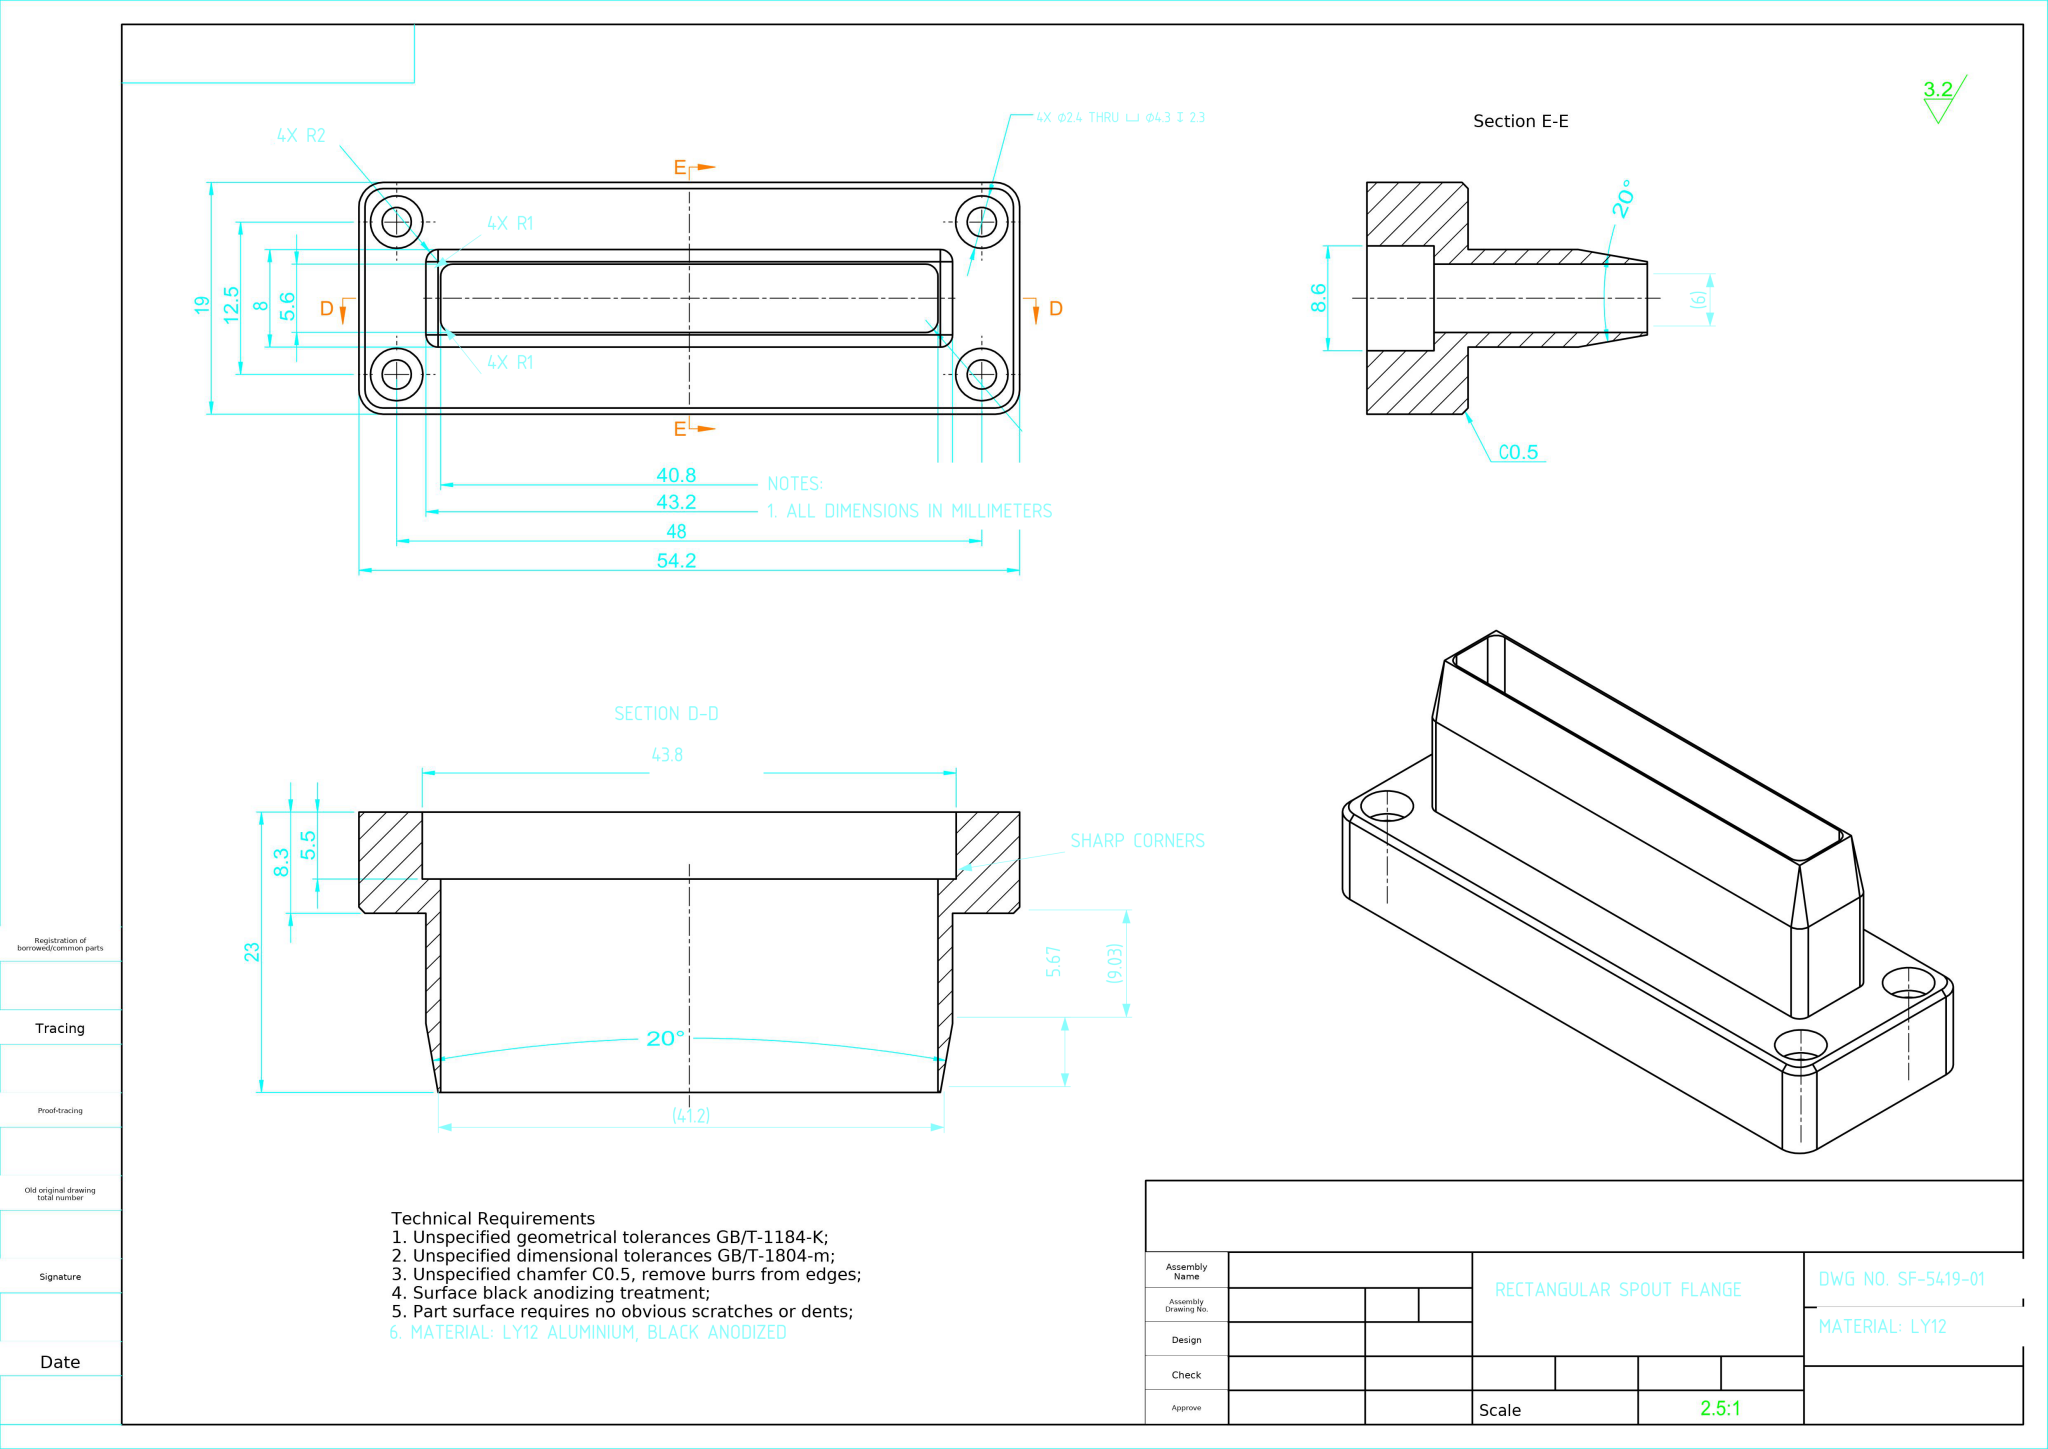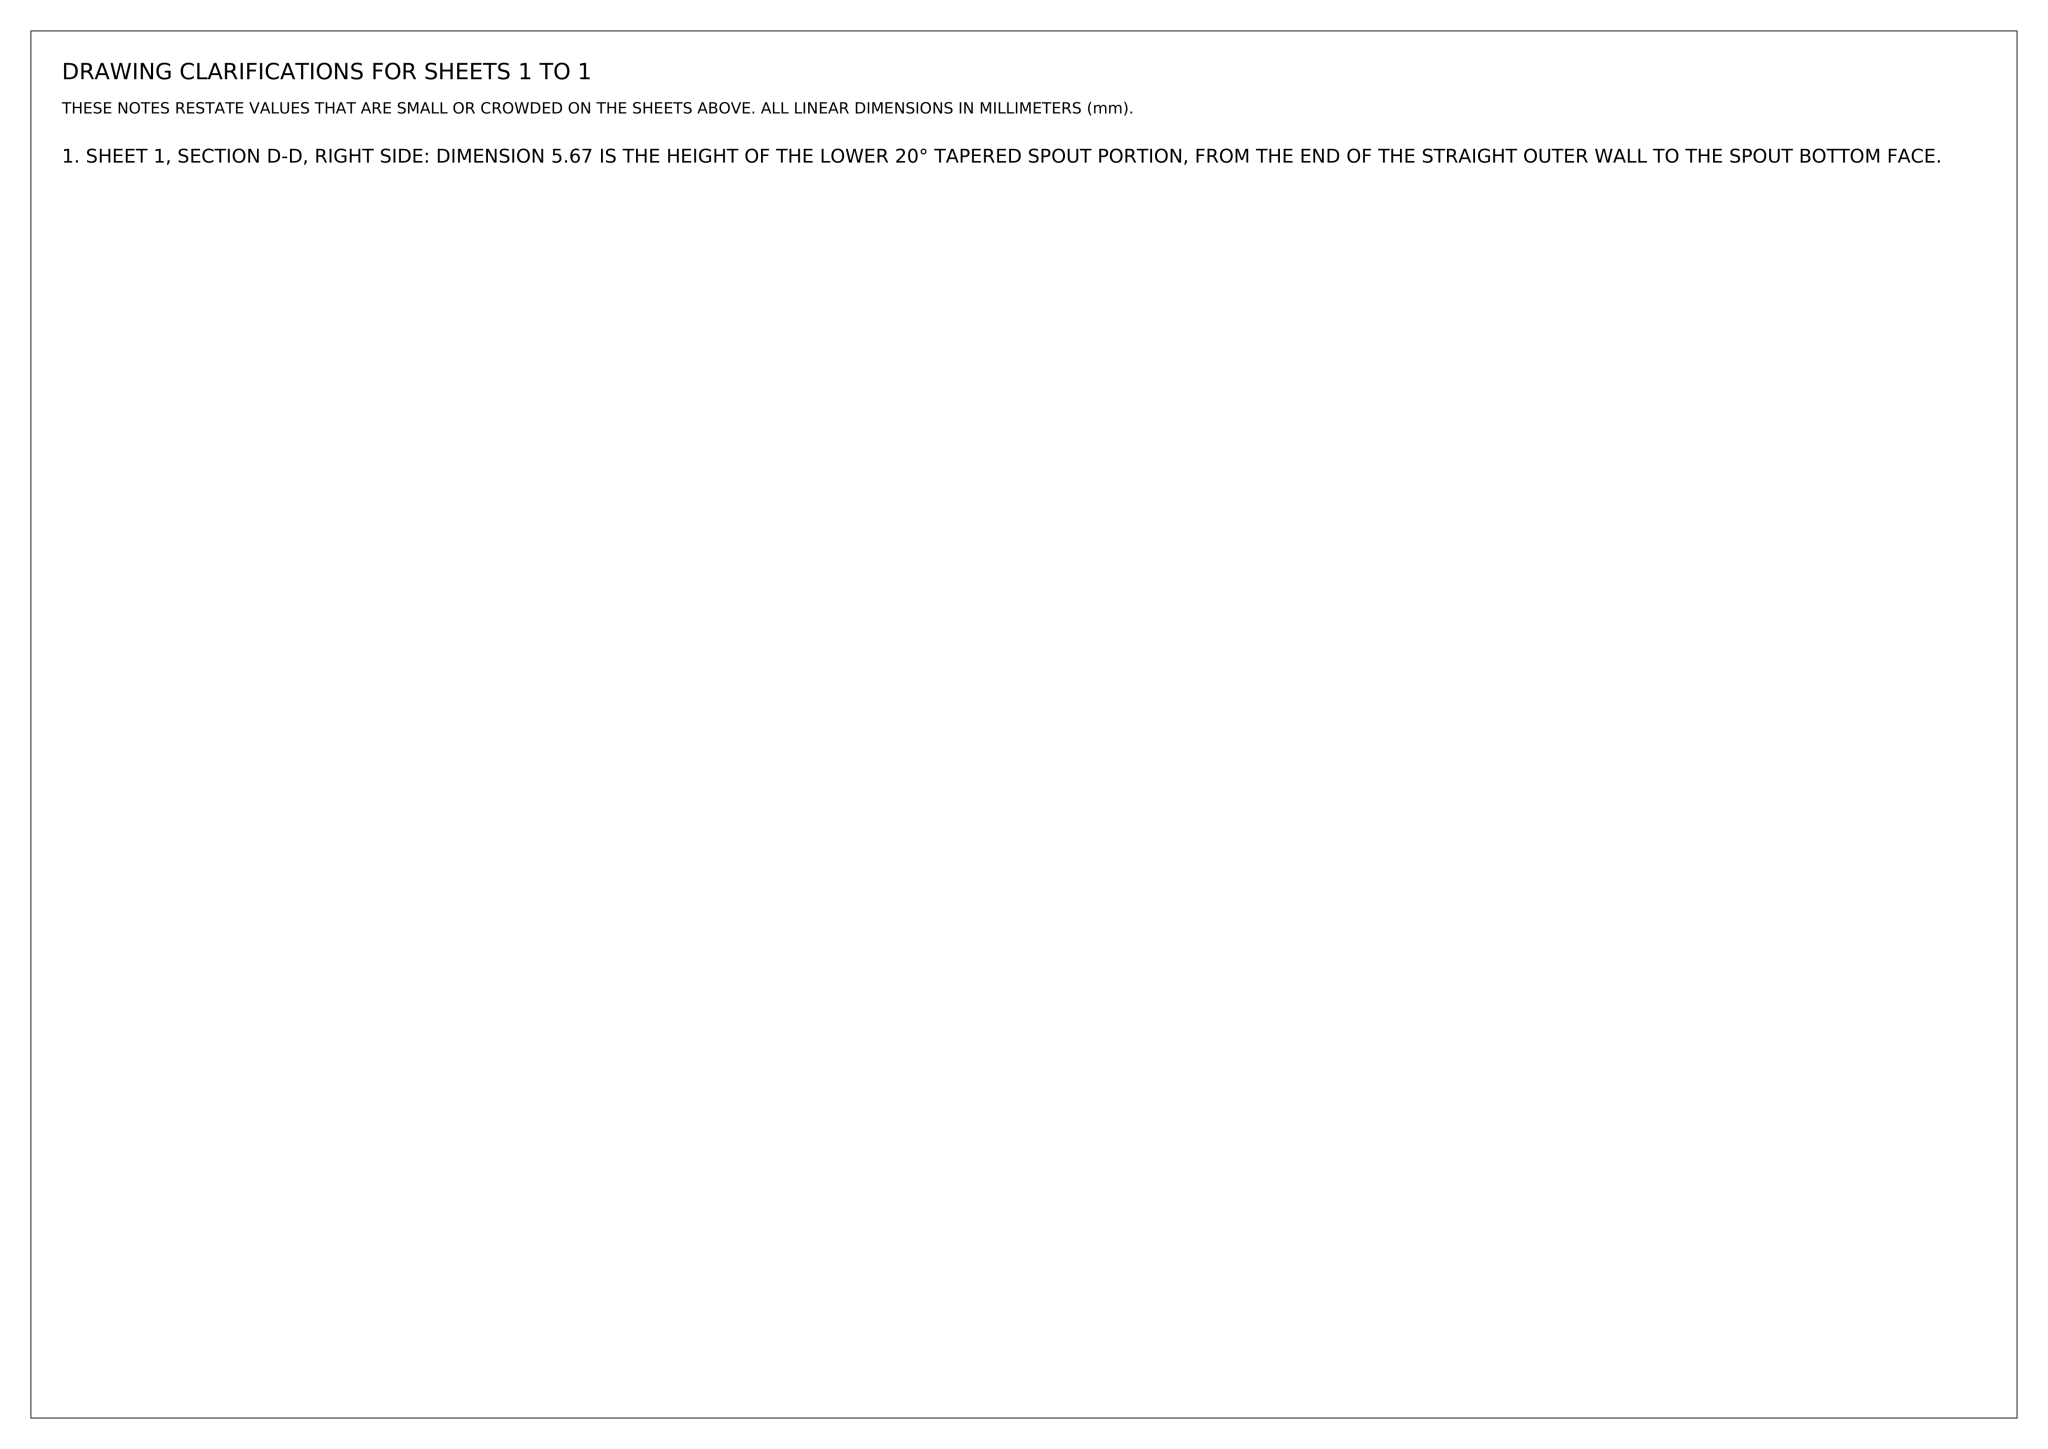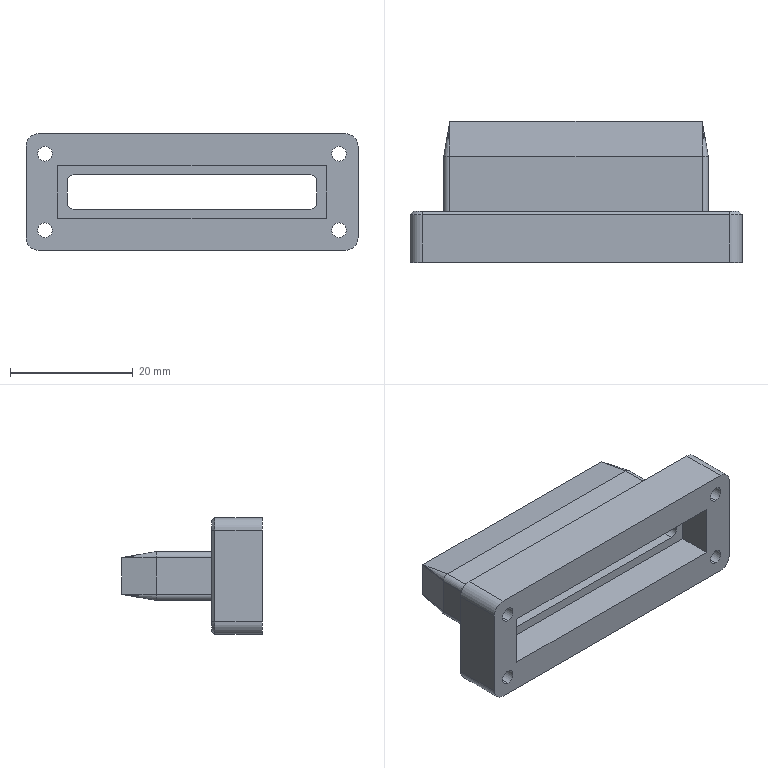Part | NX | mm | 1 solid | 68 faces | box 54.2 x 23 x 19 mm | volume 6992 mm3 | plane 32 | cylinder 28 | cone 8 | commonest cylinder face diameters 4.3 x8 2.4 x8 2 x8 4 x4